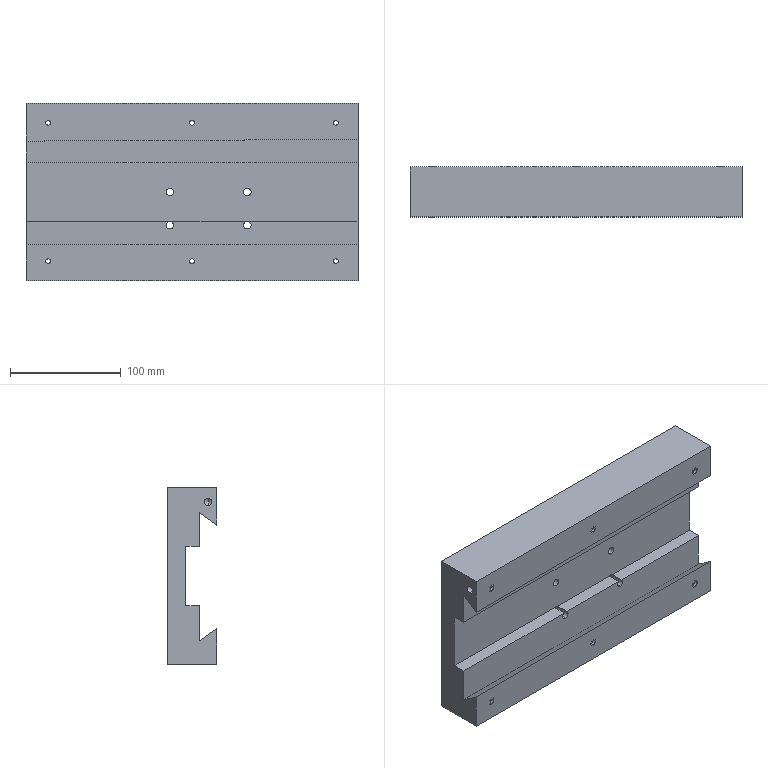Component | SolidWorks | 29SlideSeat-1 | 1 solid | 56 faces | volume 1443199 mm3 | cylinder 24 | cone 16 | plane 16 | commonest cylinder face diameters 6.8 x24